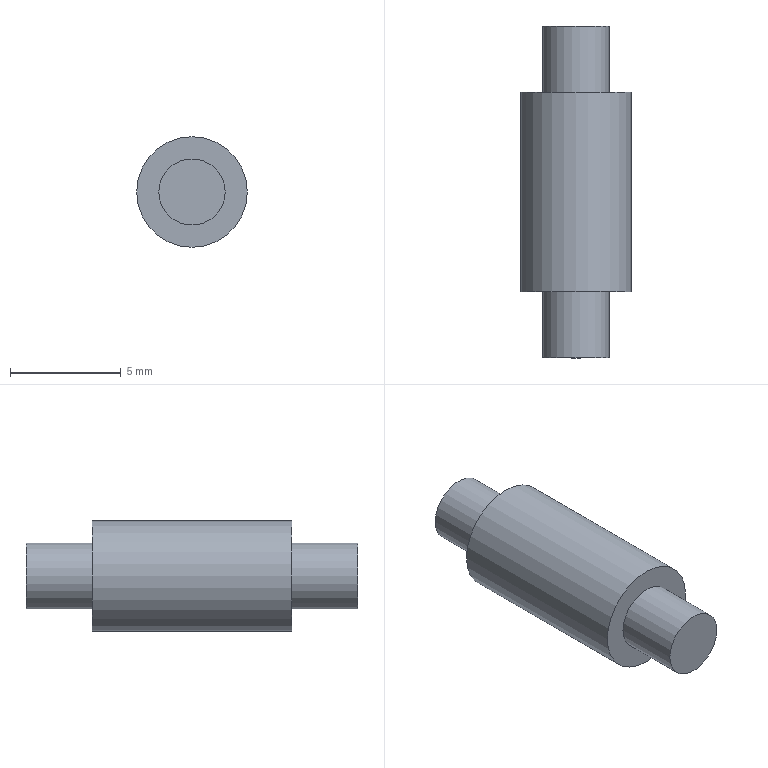Component | NX | LINK_4_PIN | 1 solid | 7 faces | volume 219 mm3 | plane 4 | cylinder 3 | commonest cylinder face diameters 3 x2 5 x1